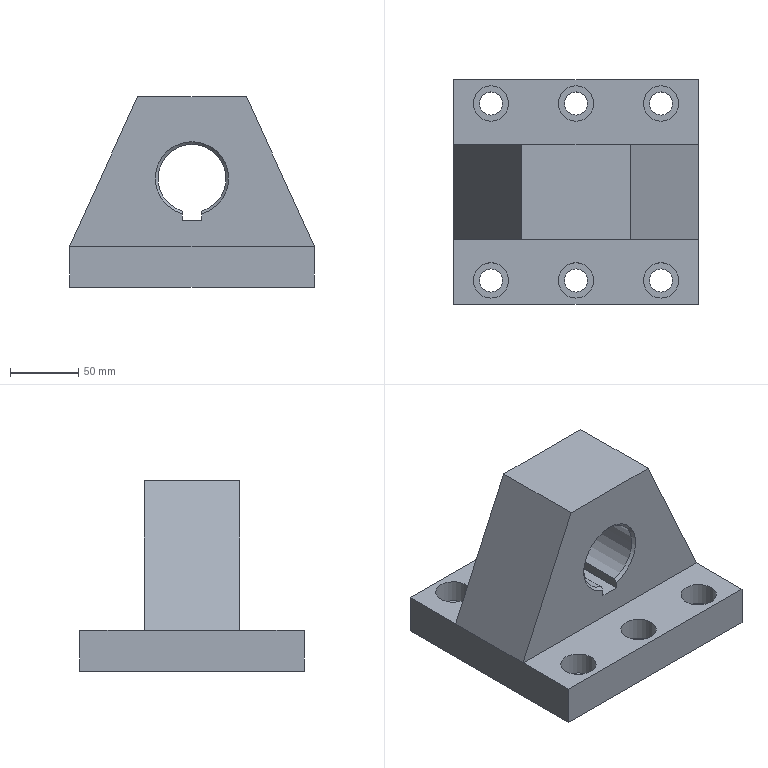Component | NX | BRACKET | 1 solid | 41 faces | volume 1664612 mm3 | plane 24 | cylinder 15 | cone 2 | commonest cylinder face diameters 17 x6 26 x6 12 x2 50 x1